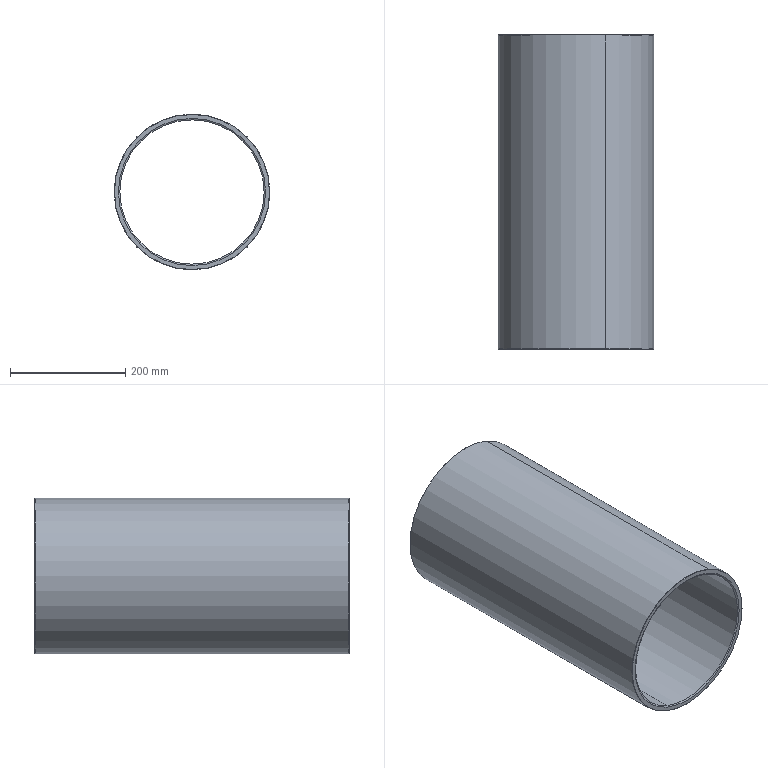Component | SolidWorks | YC1-250-04BalancerAssembly#16673-1_YC1-250-04-04CylinderBarrel#16673-1 | 1 solid | 14 faces | box 270 x 545 x 270 mm | volume 4448572 mm3 | cone 8 | cylinder 4 | plane 2 | commonest cylinder face diameters 270 x2 250 x2 | material Plain Carbon Steel
STEP:
#1=CARTESIAN_POINT('',(-13.202,157.5,-2.039));
#2=VERTEX_POINT('',#1);
#3=CARTESIAN_POINT('',(-20.149,157.5,-4.908));
#4=VERTEX_POINT('',#3);
#5=CARTESIAN_POINT('',(-18.11,157.5,0.));
#6=DIRECTION('',(-0.,1.,-0.));
#7=DIRECTION('',(0.3837,0.,0.9235));
#8=AXIS2_PLACEMENT_3D('',#5,#6,#7);
#9=CIRCLE('',#8,5.315);
#10=EDGE_CURVE('',#2,#4,#9,.T.);
#11=ORIENTED_EDGE('',*,*,#10,.T.);
#12=CARTESIAN_POINT('',(-20.149,178.917,-4.908));
#13=VERTEX_POINT('',#12);
#14=CARTESIAN_POINT('',(-20.149,157.48,-4.908));
#15=DIRECTION('',(-0.,1.,-0.));
#16=VECTOR('',#15,39.37);
#17=LINE('',#14,#16);
#18=EDGE_CURVE('',#4,#13,#17,.T.);
#19=ORIENTED_EDGE('',*,*,#18,.T.);
#20=CARTESIAN_POINT('',(-13.202,178.917,-2.039));
#21=VERTEX_POINT('',#20);
#22=CARTESIAN_POINT('',(-18.11,178.917,0.));
#23=DIRECTION('',(0.,-1.,0.));
#24=DIRECTION('',(0.3837,0.,0.9235));
#25=AXIS2_PLACEMENT_3D('',#22,#23,#24);
#26=CIRCLE('',#25,5.315);
#27=EDGE_CURVE('',#13,#21,#26,.T.);
#28=ORIENTED_EDGE('',*,*,#27,.T.);
#29=CARTESIAN_POINT('',(-16.071,178.917,4.908));
#30=VERTEX_POINT('',#29);
#31=CARTESIAN_POINT('',(-18.11,178.917,0.));
#32=DIRECTION('',(0.,-1.,0.));
#33=DIRECTION('',(0.3837,0.,0.9235));
#34=AXIS2_PLACEMENT_3D('',#31,#32,#33);
#35=CIRCLE('',#34,5.315);
#36=EDGE_CURVE('',#21,#30,#35,.T.);
#37=ORIENTED_EDGE('',*,*,#36,.T.);
#38=CARTESIAN_POINT('',(-16.071,157.5,4.908));
#39=VERTEX_POINT('',#38);
#40=CARTESIAN_POINT('',(-16.071,157.48,4.908));
#41=DIRECTION('',(-0.,1.,-0.));
#42=VECTOR('',#41,39.37);
#43=LINE('',#40,#42);
#44=EDGE_CURVE('',#39,#30,#43,.T.);
#45=ORIENTED_EDGE('',*,*,#44,.F.);
#46=CARTESIAN_POINT('',(-18.11,157.5,0.));
#47=DIRECTION('',(-0.,1.,-0.));
#48=DIRECTION('',(0.3837,0.,0.9235));
#49=AXIS2_PLACEMENT_3D('',#46,#47,#48);
#50=CIRCLE('',#49,5.315);
#51=EDGE_CURVE('',#39,#2,#50,.T.);
#52=ORIENTED_EDGE('',*,*,#51,.T.);
#53=EDGE_LOOP('',(#11,#19,#28,#37,#45,#52));
#54=FACE_OUTER_BOUND('',#53,.T.);
#55=CARTESIAN_POINT('',(-18.11,157.48,0.));
#56=DIRECTION('',(-0.,1.,-0.));
#57=DIRECTION('',(0.3837,0.,0.9235));
#58=AXIS2_PLACEMENT_3D('',#55,#56,#57);
#59=CYLINDRICAL_SURFACE('',#58,5.315);
#60=ADVANCED_FACE('',(#54),#59,.T.);
#61=CARTESIAN_POINT('',(-23.,178.937,2.032));
#62=VERTEX_POINT('',#61);
#63=CARTESIAN_POINT('',(-13.22,178.937,-2.032));
#64=VERTEX_POINT('',#63);
#65=CARTESIAN_POINT('',(-18.11,178.937,0.));
#66=DIRECTION('',(-0.,-1.,0.));
#67=DIRECTION('',(-0.9235,0.,0.3837));
#68=AXIS2_PLACEMENT_3D('',#65,#66,#67);
#69=CIRCLE('',#68,5.295);
#70=EDGE_CURVE('',#62,#64,#69,.T.);
#71=ORIENTED_EDGE('',*,*,#70,.T.);
#72=CARTESIAN_POINT('',(-13.202,178.917,-2.039));
#73=DIRECTION('',(0.653,-0.7071,-0.2713));
#74=VECTOR('',#73,39.37);
#75=LINE('',#72,#74);
#76=EDGE_CURVE('',#64,#21,#75,.T.);
#77=ORIENTED_EDGE('',*,*,#76,.T.);
#78=ORIENTED_EDGE('',*,*,#27,.F.);
#79=CARTESIAN_POINT('',(-23.018,178.917,2.039));
#80=VERTEX_POINT('',#79);
#81=CARTESIAN_POINT('',(-18.11,178.917,0.));
#82=DIRECTION('',(0.,-1.,0.));
#83=DIRECTION('',(0.3837,0.,0.9235));
#84=AXIS2_PLACEMENT_3D('',#81,#82,#83);
#85=CIRCLE('',#84,5.315);
#86=EDGE_CURVE('',#80,#13,#85,.T.);
#87=ORIENTED_EDGE('',*,*,#86,.F.);
#88=CARTESIAN_POINT('',(-23.018,178.917,2.039));
#89=DIRECTION('',(-0.653,-0.7071,0.2713));
#90=VECTOR('',#89,39.37);
#91=LINE('',#88,#90);
#92=EDGE_CURVE('',#62,#80,#91,.T.);
#93=ORIENTED_EDGE('',*,*,#92,.F.);
#94=EDGE_LOOP('',(#71,#77,#78,#87,#93));
#95=FACE_OUTER_BOUND('',#94,.T.);
#96=CARTESIAN_POINT('',(-18.11,178.917,0.));
#97=DIRECTION('',(-0.,-1.,0.));
#98=DIRECTION('',(-0.9235,0.,0.3837));
#99=AXIS2_PLACEMENT_3D('',#96,#97,#98);
#100=CONICAL_SURFACE('',#99,5.315,0.7854);
#101=ADVANCED_FACE('',(#95),#100,.T.);
#102=CARTESIAN_POINT('',(-13.22,157.48,-2.032));
#103=VERTEX_POINT('',#102);
#104=CARTESIAN_POINT('',(-23.,157.48,2.032));
#105=VERTEX_POINT('',#104);
#106=CARTESIAN_POINT('',(-18.11,157.48,0.));
#107=DIRECTION('',(-0.,1.,0.));
#108=DIRECTION('',(0.9235,0.,-0.3837));
#109=AXIS2_PLACEMENT_3D('',#106,#107,#108);
#110=CIRCLE('',#109,5.295);
#111=EDGE_CURVE('',#103,#105,#110,.T.);
#112=ORIENTED_EDGE('',*,*,#111,.T.);
#113=CARTESIAN_POINT('',(-23.018,157.5,2.039));
#114=VERTEX_POINT('',#113);
#115=CARTESIAN_POINT('',(-23.018,157.5,2.039));
#116=DIRECTION('',(-0.653,0.7071,0.2713));
#117=VECTOR('',#116,39.37);
#118=LINE('',#115,#117);
#119=EDGE_CURVE('',#105,#114,#118,.T.);
#120=ORIENTED_EDGE('',*,*,#119,.T.);
#121=CARTESIAN_POINT('',(-18.11,157.5,0.));
#122=DIRECTION('',(-0.,1.,-0.));
#123=DIRECTION('',(0.3837,0.,0.9235));
#124=AXIS2_PLACEMENT_3D('',#121,#122,#123);
#125=CIRCLE('',#124,5.315);
#126=EDGE_CURVE('',#4,#114,#125,.T.);
#127=ORIENTED_EDGE('',*,*,#126,.F.);
#128=ORIENTED_EDGE('',*,*,#10,.F.);
#129=CARTESIAN_POINT('',(-13.202,157.5,-2.039));
#130=DIRECTION('',(0.653,0.7071,-0.2713));
#131=VECTOR('',#130,39.37);
#132=LINE('',#129,#131);
#133=EDGE_CURVE('',#103,#2,#132,.T.);
#134=ORIENTED_EDGE('',*,*,#133,.F.);
#135=EDGE_LOOP('',(#112,#120,#127,#128,#134));
#136=FACE_OUTER_BOUND('',#135,.T.);
#137=CARTESIAN_POINT('',(-18.11,157.5,0.));
#138=DIRECTION('',(-0.,1.,0.));
#139=DIRECTION('',(0.9235,0.,-0.3837));
#140=AXIS2_PLACEMENT_3D('',#137,#138,#139);
#141=CONICAL_SURFACE('',#140,5.315,0.7854);
#142=ADVANCED_FACE('',(#136),#141,.T.);
#143=CARTESIAN_POINT('',(-19.998,178.88,-4.545));
#144=VERTEX_POINT('',#143);
#145=CARTESIAN_POINT('',(-16.222,178.88,4.545));
#146=VERTEX_POINT('',#145);
#147=CARTESIAN_POINT('',(-18.11,178.88,0.));
#148=DIRECTION('',(-0.,1.,-0.));
#149=DIRECTION('',(0.3837,0.,0.9235));
#150=AXIS2_PLACEMENT_3D('',#147,#148,#149);
#151=CIRCLE('',#150,4.921);
#152=EDGE_CURVE('',#144,#146,#151,.T.);
#153=ORIENTED_EDGE('',*,*,#152,.F.);
#154=CARTESIAN_POINT('',(-20.036,178.937,-4.636));
#155=VERTEX_POINT('',#154);
#156=CARTESIAN_POINT('',(-20.036,178.937,-4.636));
#157=DIRECTION('',(-0.3323,0.5,-0.7997));
#158=VECTOR('',#157,39.37);
#159=LINE('',#156,#158);
#160=EDGE_CURVE('',#144,#155,#159,.T.);
#161=ORIENTED_EDGE('',*,*,#160,.T.);
#162=CARTESIAN_POINT('',(-16.184,178.937,4.636));
#163=VERTEX_POINT('',#162);
#164=CARTESIAN_POINT('',(-18.11,178.937,0.));
#165=DIRECTION('',(-0.,1.,-0.));
#166=DIRECTION('',(0.3837,0.,0.9235));
#167=AXIS2_PLACEMENT_3D('',#164,#165,#166);
#168=CIRCLE('',#167,5.02);
#169=EDGE_CURVE('',#155,#163,#168,.T.);
#170=ORIENTED_EDGE('',*,*,#169,.T.);
#171=CARTESIAN_POINT('',(-16.184,178.937,4.636));
#172=DIRECTION('',(0.3323,0.5,0.7997));
#173=VECTOR('',#172,39.37);
#174=LINE('',#171,#173);
#175=EDGE_CURVE('',#146,#163,#174,.T.);
#176=ORIENTED_EDGE('',*,*,#175,.F.);
#177=EDGE_LOOP('',(#153,#161,#170,#176));
#178=FACE_OUTER_BOUND('',#177,.T.);
#179=CARTESIAN_POINT('',(-18.11,178.937,0.));
#180=DIRECTION('',(-0.,1.,-0.));
#181=DIRECTION('',(0.3837,0.,0.9235));
#182=AXIS2_PLACEMENT_3D('',#179,#180,#181);
#183=CONICAL_SURFACE('',#182,5.02,1.047);
#184=ADVANCED_FACE('',(#178),#183,.F.);
#185=CARTESIAN_POINT('',(-16.222,157.537,4.545));
#186=VERTEX_POINT('',#185);
#187=CARTESIAN_POINT('',(-19.998,157.537,-4.545));
#188=VERTEX_POINT('',#187);
#189=CARTESIAN_POINT('',(-18.11,157.537,0.));
#190=DIRECTION('',(0.,-1.,0.));
#191=DIRECTION('',(-0.3837,0.,-0.9235));
#192=AXIS2_PLACEMENT_3D('',#189,#190,#191);
#193=CIRCLE('',#192,4.921);
#194=EDGE_CURVE('',#186,#188,#193,.T.);
#195=ORIENTED_EDGE('',*,*,#194,.F.);
#196=CARTESIAN_POINT('',(-16.184,157.48,4.636));
#197=VERTEX_POINT('',#196);
#198=CARTESIAN_POINT('',(-16.184,157.48,4.636));
#199=DIRECTION('',(0.3323,-0.5,0.7997));
#200=VECTOR('',#199,39.37);
#201=LINE('',#198,#200);
#202=EDGE_CURVE('',#186,#197,#201,.T.);
#203=ORIENTED_EDGE('',*,*,#202,.T.);
#204=CARTESIAN_POINT('',(-20.036,157.48,-4.636));
#205=VERTEX_POINT('',#204);
#206=CARTESIAN_POINT('',(-18.11,157.48,0.));
#207=DIRECTION('',(-0.,1.,-0.));
#208=DIRECTION('',(-0.3837,0.,-0.9235));
#209=AXIS2_PLACEMENT_3D('',#206,#207,#208);
#210=CIRCLE('',#209,5.02);
#211=EDGE_CURVE('',#205,#197,#210,.T.);
#212=ORIENTED_EDGE('',*,*,#211,.F.);
#213=CARTESIAN_POINT('',(-20.036,157.48,-4.636));
#214=DIRECTION('',(-0.3323,-0.5,-0.7997));
#215=VECTOR('',#214,39.37);
#216=LINE('',#213,#215);
#217=EDGE_CURVE('',#188,#205,#216,.T.);
#218=ORIENTED_EDGE('',*,*,#217,.F.);
#219=EDGE_LOOP('',(#195,#203,#212,#218));
#220=FACE_OUTER_BOUND('',#219,.T.);
#221=CARTESIAN_POINT('',(-18.11,157.48,0.));
#222=DIRECTION('',(0.,-1.,0.));
#223=DIRECTION('',(-0.3837,0.,-0.9235));
#224=AXIS2_PLACEMENT_3D('',#221,#222,#223);
#225=CONICAL_SURFACE('',#224,5.02,1.047);
#226=ADVANCED_FACE('',(#220),#225,.F.);
#227=ORIENTED_EDGE('',*,*,#194,.T.);
#228=CARTESIAN_POINT('',(-19.998,157.48,-4.545));
#229=DIRECTION('',(-0.,1.,-0.));
#230=VECTOR('',#229,39.37);
#231=LINE('',#228,#230);
#232=EDGE_CURVE('',#188,#144,#231,.T.);
#233=ORIENTED_EDGE('',*,*,#232,.T.);
#234=ORIENTED_EDGE('',*,*,#152,.T.);
#235=CARTESIAN_POINT('',(-16.222,157.48,4.545));
#236=DIRECTION('',(-0.,1.,-0.));
#237=VECTOR('',#236,39.37);
#238=LINE('',#235,#237);
#239=EDGE_CURVE('',#186,#146,#238,.T.);
#240=ORIENTED_EDGE('',*,*,#239,.F.);
#241=EDGE_LOOP('',(#227,#233,#234,#240));
#242=FACE_OUTER_BOUND('',#241,.T.);
#243=CARTESIAN_POINT('',(-18.11,157.48,0.));
#244=DIRECTION('',(-0.,1.,-0.));
#245=DIRECTION('',(0.3837,0.,0.9235));
#246=AXIS2_PLACEMENT_3D('',#243,#244,#245);
#247=CYLINDRICAL_SURFACE('',#246,4.921);
#248=ADVANCED_FACE('',(#242),#247,.F.);
#249=ORIENTED_EDGE('',*,*,#18,.F.);
#250=ORIENTED_EDGE('',*,*,#126,.T.);
#251=CARTESIAN_POINT('',(-18.11,157.5,0.));
#252=DIRECTION('',(-0.,1.,-0.));
#253=DIRECTION('',(0.3837,0.,0.9235));
#254=AXIS2_PLACEMENT_3D('',#251,#252,#253);
#255=CIRCLE('',#254,5.315);
#256=EDGE_CURVE('',#114,#39,#255,.T.);
#257=ORIENTED_EDGE('',*,*,#256,.T.);
#258=ORIENTED_EDGE('',*,*,#44,.T.);
#259=CARTESIAN_POINT('',(-18.11,178.917,0.));
#260=DIRECTION('',(0.,-1.,0.));
#261=DIRECTION('',(0.3837,0.,0.9235));
#262=AXIS2_PLACEMENT_3D('',#259,#260,#261);
#263=CIRCLE('',#262,5.315);
#264=EDGE_CURVE('',#30,#80,#263,.T.);
#265=ORIENTED_EDGE('',*,*,#264,.T.);
#266=ORIENTED_EDGE('',*,*,#86,.T.);
#267=EDGE_LOOP('',(#249,#250,#257,#258,#265,#266));
#268=FACE_OUTER_BOUND('',#267,.T.);
#269=CARTESIAN_POINT('',(-18.11,157.48,0.));
#270=DIRECTION('',(-0.,1.,-0.));
#271=DIRECTION('',(0.3837,0.,0.9235));
#272=AXIS2_PLACEMENT_3D('',#269,#270,#271);
#273=CYLINDRICAL_SURFACE('',#272,5.315);
#274=ADVANCED_FACE('',(#268),#273,.T.);
#275=ORIENTED_EDGE('',*,*,#76,.F.);
#276=CARTESIAN_POINT('',(-18.11,178.937,0.));
#277=DIRECTION('',(-0.,-1.,0.));
#278=DIRECTION('',(-0.9235,0.,0.3837));
#279=AXIS2_PLACEMENT_3D('',#276,#277,#278);
#280=CIRCLE('',#279,5.295);
#281=EDGE_CURVE('',#64,#62,#280,.T.);
#282=ORIENTED_EDGE('',*,*,#281,.T.);
#283=ORIENTED_EDGE('',*,*,#92,.T.);
#284=ORIENTED_EDGE('',*,*,#264,.F.);
#285=ORIENTED_EDGE('',*,*,#36,.F.);
#286=EDGE_LOOP('',(#275,#282,#283,#284,#285));
#287=FACE_OUTER_BOUND('',#286,.T.);
#288=CARTESIAN_POINT('',(-18.11,178.917,0.));
#289=DIRECTION('',(-0.,-1.,0.));
#290=DIRECTION('',(-0.9235,0.,0.3837));
#291=AXIS2_PLACEMENT_3D('',#288,#289,#290);
#292=CONICAL_SURFACE('',#291,5.315,0.7854);
#293=ADVANCED_FACE('',(#287),#292,.T.);
#294=ORIENTED_EDGE('',*,*,#119,.F.);
#295=CARTESIAN_POINT('',(-18.11,157.48,0.));
#296=DIRECTION('',(-0.,1.,0.));
#297=DIRECTION('',(0.9235,0.,-0.3837));
#298=AXIS2_PLACEMENT_3D('',#295,#296,#297);
#299=CIRCLE('',#298,5.295);
#300=EDGE_CURVE('',#105,#103,#299,.T.);
#301=ORIENTED_EDGE('',*,*,#300,.T.);
#302=ORIENTED_EDGE('',*,*,#133,.T.);
#303=ORIENTED_EDGE('',*,*,#51,.F.);
#304=ORIENTED_EDGE('',*,*,#256,.F.);
#305=EDGE_LOOP('',(#294,#301,#302,#303,#304));
#306=FACE_OUTER_BOUND('',#305,.T.);
#307=CARTESIAN_POINT('',(-18.11,157.5,0.));
#308=DIRECTION('',(-0.,1.,0.));
#309=DIRECTION('',(0.9235,0.,-0.3837));
#310=AXIS2_PLACEMENT_3D('',#307,#308,#309);
#311=CONICAL_SURFACE('',#310,5.315,0.7854);
#312=ADVANCED_FACE('',(#306),#311,.T.);
#313=ORIENTED_EDGE('',*,*,#70,.F.);
#314=ORIENTED_EDGE('',*,*,#281,.F.);
#315=EDGE_LOOP('',(#313,#314));
#316=FACE_OUTER_BOUND('',#315,.T.);
#317=CARTESIAN_POINT('',(-18.11,178.937,0.));
#318=DIRECTION('',(-0.,1.,-0.));
#319=DIRECTION('',(0.3837,0.,0.9235));
#320=AXIS2_PLACEMENT_3D('',#317,#318,#319);
#321=CIRCLE('',#320,5.02);
#322=EDGE_CURVE('',#163,#155,#321,.T.);
#323=ORIENTED_EDGE('',*,*,#322,.F.);
#324=ORIENTED_EDGE('',*,*,#169,.F.);
#325=EDGE_LOOP('',(#323,#324));
#326=FACE_BOUND('',#325,.T.);
#327=CARTESIAN_POINT('',(-18.11,178.937,0.));
#328=DIRECTION('',(0.,-1.,0.));
#329=DIRECTION('',(-0.3837,-0.,-0.9235));
#330=AXIS2_PLACEMENT_3D('',#327,#328,#329);
#331=PLANE('',#330);
#332=ADVANCED_FACE('',(#316,#326),#331,.F.);
#333=ORIENTED_EDGE('',*,*,#111,.F.);
#334=ORIENTED_EDGE('',*,*,#300,.F.);
#335=EDGE_LOOP('',(#333,#334));
#336=FACE_OUTER_BOUND('',#335,.T.);
#337=ORIENTED_EDGE('',*,*,#211,.T.);
#338=CARTESIAN_POINT('',(-18.11,157.48,0.));
#339=DIRECTION('',(-0.,1.,-0.));
#340=DIRECTION('',(-0.3837,0.,-0.9235));
#341=AXIS2_PLACEMENT_3D('',#338,#339,#340);
#342=CIRCLE('',#341,5.02);
#343=EDGE_CURVE('',#197,#205,#342,.T.);
#344=ORIENTED_EDGE('',*,*,#343,.T.);
#345=EDGE_LOOP('',(#337,#344));
#346=FACE_BOUND('',#345,.T.);
#347=CARTESIAN_POINT('',(-18.11,157.48,0.));
#348=DIRECTION('',(0.,-1.,0.));
#349=DIRECTION('',(-0.3837,-0.,-0.9235));
#350=AXIS2_PLACEMENT_3D('',#347,#348,#349);
#351=PLANE('',#350);
#352=ADVANCED_FACE('',(#336,#346),#351,.T.);
#353=ORIENTED_EDGE('',*,*,#160,.F.);
#354=CARTESIAN_POINT('',(-18.11,178.88,0.));
#355=DIRECTION('',(-0.,1.,-0.));
#356=DIRECTION('',(0.3837,0.,0.9235));
#357=AXIS2_PLACEMENT_3D('',#354,#355,#356);
#358=CIRCLE('',#357,4.921);
#359=EDGE_CURVE('',#146,#144,#358,.T.);
#360=ORIENTED_EDGE('',*,*,#359,.F.);
#361=ORIENTED_EDGE('',*,*,#175,.T.);
#362=ORIENTED_EDGE('',*,*,#322,.T.);
#363=EDGE_LOOP('',(#353,#360,#361,#362));
#364=FACE_OUTER_BOUND('',#363,.T.);
#365=CARTESIAN_POINT('',(-18.11,178.937,0.));
#366=DIRECTION('',(-0.,1.,-0.));
#367=DIRECTION('',(0.3837,0.,0.9235));
#368=AXIS2_PLACEMENT_3D('',#365,#366,#367);
#369=CONICAL_SURFACE('',#368,5.02,1.047);
#370=ADVANCED_FACE('',(#364),#369,.F.);
#371=ORIENTED_EDGE('',*,*,#202,.F.);
#372=CARTESIAN_POINT('',(-18.11,157.537,0.));
#373=DIRECTION('',(0.,-1.,0.));
#374=DIRECTION('',(-0.3837,0.,-0.9235));
#375=AXIS2_PLACEMENT_3D('',#372,#373,#374);
#376=CIRCLE('',#375,4.921);
#377=EDGE_CURVE('',#188,#186,#376,.T.);
#378=ORIENTED_EDGE('',*,*,#377,.F.);
#379=ORIENTED_EDGE('',*,*,#217,.T.);
#380=ORIENTED_EDGE('',*,*,#343,.F.);
#381=EDGE_LOOP('',(#371,#378,#379,#380));
#382=FACE_OUTER_BOUND('',#381,.T.);
#383=CARTESIAN_POINT('',(-18.11,157.48,0.));
#384=DIRECTION('',(0.,-1.,0.));
#385=DIRECTION('',(-0.3837,0.,-0.9235));
#386=AXIS2_PLACEMENT_3D('',#383,#384,#385);
#387=CONICAL_SURFACE('',#386,5.02,1.047);
#388=ADVANCED_FACE('',(#382),#387,.F.);
#389=ORIENTED_EDGE('',*,*,#232,.F.);
#390=ORIENTED_EDGE('',*,*,#377,.T.);
#391=ORIENTED_EDGE('',*,*,#239,.T.);
#392=ORIENTED_EDGE('',*,*,#359,.T.);
#393=EDGE_LOOP('',(#389,#390,#391,#392));
#394=FACE_OUTER_BOUND('',#393,.T.);
#395=CARTESIAN_POINT('',(-18.11,157.48,0.));
#396=DIRECTION('',(-0.,1.,-0.));
#397=DIRECTION('',(0.3837,0.,0.9235));
#398=AXIS2_PLACEMENT_3D('',#395,#396,#397);
#399=CYLINDRICAL_SURFACE('',#398,4.921);
#400=ADVANCED_FACE('',(#394),#399,.F.);
#401=CLOSED_SHELL('',(#60,#101,#142,#184,#226,#248,#274,#293,#312,#332,#352,#370,#388,#400));
#402=MANIFOLD_SOLID_BREP('',#401);
#403=CARTESIAN_POINT('',(0.,0.,0.));
#404=DIRECTION('',(0.,0.,1.));
#405=DIRECTION('',(1.,0.,0.));
#406=AXIS2_PLACEMENT_3D('',#403,#404,#405);
#407=(LENGTH_UNIT()NAMED_UNIT(*)SI_UNIT($,.METRE.));
#408=LENGTH_MEASURE_WITH_UNIT(LENGTH_MEASURE(0.0254),#407);
#409=DIMENSIONAL_EXPONENTS(1.,0.,0.,0.,0.,0.,0.);
#410=(CONVERSION_BASED_UNIT('',#408)LENGTH_UNIT()NAMED_UNIT(#409));
#411=UNCERTAINTY_MEASURE_WITH_UNIT(LENGTH_MEASURE(0.00001),#410,'','');
#412=(NAMED_UNIT(*)PLANE_ANGLE_UNIT()SI_UNIT($,.RADIAN.));
#413=(NAMED_UNIT(*)SI_UNIT($,.STERADIAN.)SOLID_ANGLE_UNIT());
#414=(GEOMETRIC_REPRESENTATION_CONTEXT(3)GLOBAL_UNCERTAINTY_ASSIGNED_CONTEXT((#411))GLOBAL_UNIT_ASSIGNED_CONTEXT((#410,#412,#413))REPRESENTATION_CONTEXT('',''));
#415=ADVANCED_BREP_SHAPE_REPRESENTATION('',(#402,#406),#414);
#416=COLOUR_RGB('',0.7922,0.8196,0.9333);
#417=FILL_AREA_STYLE_COLOUR('',#416);
#418=FILL_AREA_STYLE('',(#417));
#419=SURFACE_STYLE_FILL_AREA(#418);
#420=SURFACE_SIDE_STYLE('',(#419));
#421=SURFACE_STYLE_USAGE(.BOTH.,#420);
#422=PRESENTATION_STYLE_ASSIGNMENT((#421));
#423=STYLED_ITEM('',(#422),#402);
#424=PRESENTATION_LAYER_ASSIGNMENT('','',(#423));
#425=(LENGTH_UNIT()NAMED_UNIT(*)SI_UNIT($,.METRE.));
#426=LENGTH_MEASURE_WITH_UNIT(LENGTH_MEASURE(0.0254),#425);
#427=DIMENSIONAL_EXPONENTS(1.,0.,0.,0.,0.,0.,0.);
#428=(CONVERSION_BASED_UNIT('',#426)LENGTH_UNIT()NAMED_UNIT(#427));
#429=UNCERTAINTY_MEASURE_WITH_UNIT(LENGTH_MEASURE(0.00001),#428,'','');
#430=(NAMED_UNIT(*)PLANE_ANGLE_UNIT()SI_UNIT($,.RADIAN.));
#431=(NAMED_UNIT(*)SI_UNIT($,.STERADIAN.)SOLID_ANGLE_UNIT());
#432=(GEOMETRIC_REPRESENTATION_CONTEXT(3)GLOBAL_UNCERTAINTY_ASSIGNED_CONTEXT((#429))GLOBAL_UNIT_ASSIGNED_CONTEXT((#428,#430,#431))REPRESENTATION_CONTEXT('',''));
#433=MECHANICAL_DESIGN_GEOMETRIC_PRESENTATION_REPRESENTATION('',(#423),#432);